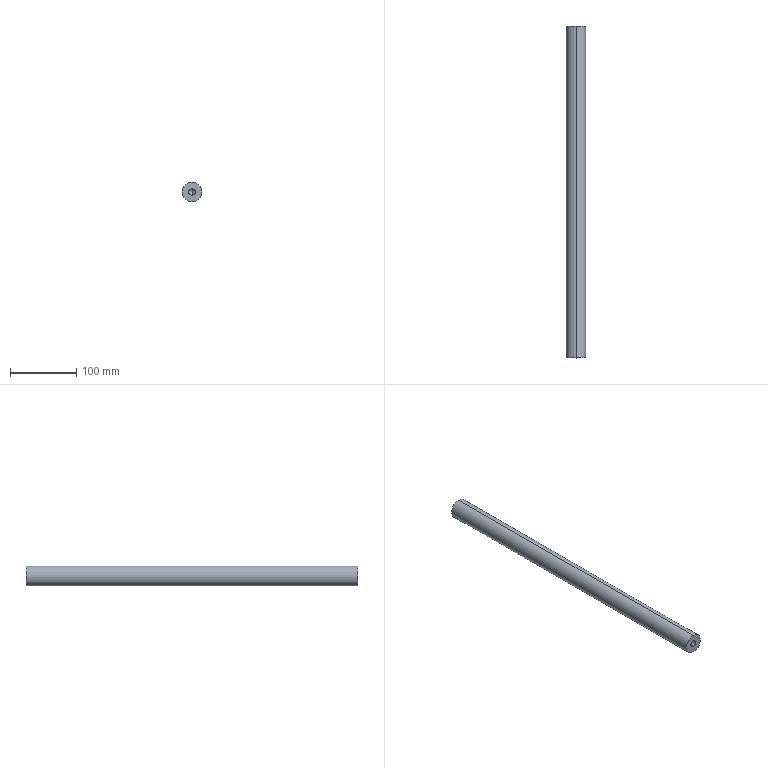Component | SolidWorks | -TopPlateSupport-1 | 1 solid | 12 faces | box 30 x 500 x 30 mm | volume 347910 mm3 | cylinder 6 | cone 4 | plane 2 | commonest cylinder face diameters 10.2 x4 30 x2
build123d program:
from build123d import *

# Parameters (mm, degrees)
SKETCH1_R           = 15
BOSS_EXTRUDE1_DEPTH = 250


with BuildPart() as part:
    # Sketch1 → Boss-Extrude1 (new, symmetric)
    with BuildSketch(Plane(origin=(0, 0, 0), x_dir=(1, 0, 0), z_dir=(0, 1, 0))):
        with Locations(Location((0, 0, 0), (0, 0, 270))):
            Circle(SKETCH1_R)
    extrude(amount=BOSS_EXTRUDE1_DEPTH, both=True)

    # Sketch2 → M12 Tapped Hole1 (revolve, cut)
    with BuildSketch(Plane(origin=(0, 250, 0), x_dir=(0, 0, 1), z_dir=(1, 0, 0))):
        Polygon((0, 0), (0, 35.814), (5.1, 32.75), (5.1, 0), align=None)
    m12_tapped_hole1 = revolve(axis=Axis((0, 256.35, 0), (0, -1, 0)), mode=Mode.SUBTRACT)

    # Mirror1: M12 Tapped Hole1 across plane
    add(m12_tapped_hole1.mirror(Plane.ZX), mode=Mode.SUBTRACT)


solid = part.part

# Placed as in the assembly
solid = solid.moved(Location((130, 1186, -180), (0, 0, 0)))
STEP:
#1=CARTESIAN_POINT('',(5.118,38.14,-6.886));
#2=VERTEX_POINT('',#1);
#3=CARTESIAN_POINT('',(5.118,38.14,-7.287));
#4=VERTEX_POINT('',#3);
#5=CARTESIAN_POINT('',(5.118,38.14,-7.087));
#6=DIRECTION('',(0.,-1.,0.));
#7=DIRECTION('',(0.,0.,-1.));
#8=AXIS2_PLACEMENT_3D('',#5,#6,#7);
#9=CIRCLE('',#8,0.2008);
#10=EDGE_CURVE('',#2,#4,#9,.T.);
#11=ORIENTED_EDGE('',*,*,#10,.F.);
#12=CARTESIAN_POINT('',(5.118,36.85,-6.886));
#13=VERTEX_POINT('',#12);
#14=CARTESIAN_POINT('',(5.118,36.85,-6.886));
#15=DIRECTION('',(0.,-1.,0.));
#16=VECTOR('',#15,39.37);
#17=LINE('',#14,#16);
#18=EDGE_CURVE('',#2,#13,#17,.T.);
#19=ORIENTED_EDGE('',*,*,#18,.T.);
#20=CARTESIAN_POINT('',(5.118,36.85,-7.287));
#21=VERTEX_POINT('',#20);
#22=CARTESIAN_POINT('',(5.118,36.85,-7.087));
#23=DIRECTION('',(0.,-1.,0.));
#24=DIRECTION('',(0.,0.,-1.));
#25=AXIS2_PLACEMENT_3D('',#22,#23,#24);
#26=CIRCLE('',#25,0.2008);
#27=EDGE_CURVE('',#13,#21,#26,.T.);
#28=ORIENTED_EDGE('',*,*,#27,.T.);
#29=CARTESIAN_POINT('',(5.118,36.85,-7.287));
#30=DIRECTION('',(0.,-1.,0.));
#31=VECTOR('',#30,39.37);
#32=LINE('',#29,#31);
#33=EDGE_CURVE('',#4,#21,#32,.T.);
#34=ORIENTED_EDGE('',*,*,#33,.F.);
#35=EDGE_LOOP('',(#11,#19,#28,#34));
#36=FACE_OUTER_BOUND('',#35,.T.);
#37=CARTESIAN_POINT('',(5.118,36.85,-7.087));
#38=DIRECTION('',(0.,-1.,0.));
#39=DIRECTION('',(0.,0.,-1.));
#40=AXIS2_PLACEMENT_3D('',#37,#38,#39);
#41=CYLINDRICAL_SURFACE('',#40,0.2008);
#42=ADVANCED_FACE('',(#36),#41,.F.);
#43=CARTESIAN_POINT('',(5.118,38.26,-7.087));
#44=VERTEX_POINT('',#43);
#45=CARTESIAN_POINT('',(5.118,38.14,-7.287));
#46=DIRECTION('',(0.,-0.515,-0.8572));
#47=VECTOR('',#46,39.37);
#48=LINE('',#45,#47);
#49=EDGE_CURVE('',#44,#4,#48,.T.);
#50=ORIENTED_EDGE('',*,*,#49,.F.);
#51=CARTESIAN_POINT('',(5.118,38.14,-6.886));
#52=DIRECTION('',(0.,-0.515,0.8572));
#53=VECTOR('',#52,39.37);
#54=LINE('',#51,#53);
#55=EDGE_CURVE('',#44,#2,#54,.T.);
#56=ORIENTED_EDGE('',*,*,#55,.T.);
#57=ORIENTED_EDGE('',*,*,#10,.T.);
#58=EDGE_LOOP('',(#50,#56,#57));
#59=FACE_OUTER_BOUND('',#58,.T.);
#60=CARTESIAN_POINT('',(5.118,38.14,-7.087));
#61=DIRECTION('',(0.,-1.,0.));
#62=DIRECTION('',(0.,0.,-1.));
#63=AXIS2_PLACEMENT_3D('',#60,#61,#62);
#64=CONICAL_SURFACE('',#63,0.2008,1.03);
#65=ADVANCED_FACE('',(#59),#64,.F.);
#66=CARTESIAN_POINT('',(5.118,55.246,-7.287));
#67=VERTEX_POINT('',#66);
#68=CARTESIAN_POINT('',(5.118,55.246,-6.886));
#69=VERTEX_POINT('',#68);
#70=CARTESIAN_POINT('',(5.118,55.246,-7.087));
#71=DIRECTION('',(0.,1.,0.));
#72=DIRECTION('',(0.,0.,1.));
#73=AXIS2_PLACEMENT_3D('',#70,#71,#72);
#74=CIRCLE('',#73,0.2008);
#75=EDGE_CURVE('',#67,#69,#74,.T.);
#76=ORIENTED_EDGE('',*,*,#75,.F.);
#77=CARTESIAN_POINT('',(5.118,56.535,-7.287));
#78=VERTEX_POINT('',#77);
#79=CARTESIAN_POINT('',(5.118,56.535,-7.287));
#80=DIRECTION('',(0.,1.,0.));
#81=VECTOR('',#80,39.37);
#82=LINE('',#79,#81);
#83=EDGE_CURVE('',#67,#78,#82,.T.);
#84=ORIENTED_EDGE('',*,*,#83,.T.);
#85=CARTESIAN_POINT('',(5.118,56.535,-6.886));
#86=VERTEX_POINT('',#85);
#87=CARTESIAN_POINT('',(5.118,56.535,-7.087));
#88=DIRECTION('',(0.,1.,0.));
#89=DIRECTION('',(0.,0.,1.));
#90=AXIS2_PLACEMENT_3D('',#87,#88,#89);
#91=CIRCLE('',#90,0.2008);
#92=EDGE_CURVE('',#78,#86,#91,.T.);
#93=ORIENTED_EDGE('',*,*,#92,.T.);
#94=CARTESIAN_POINT('',(5.118,56.535,-6.886));
#95=DIRECTION('',(0.,1.,0.));
#96=VECTOR('',#95,39.37);
#97=LINE('',#94,#96);
#98=EDGE_CURVE('',#69,#86,#97,.T.);
#99=ORIENTED_EDGE('',*,*,#98,.F.);
#100=EDGE_LOOP('',(#76,#84,#93,#99));
#101=FACE_OUTER_BOUND('',#100,.T.);
#102=CARTESIAN_POINT('',(5.118,56.535,-7.087));
#103=DIRECTION('',(0.,1.,0.));
#104=DIRECTION('',(0.,0.,1.));
#105=AXIS2_PLACEMENT_3D('',#102,#103,#104);
#106=CYLINDRICAL_SURFACE('',#105,0.2008);
#107=ADVANCED_FACE('',(#101),#106,.F.);
#108=CARTESIAN_POINT('',(5.118,55.125,-7.087));
#109=VERTEX_POINT('',#108);
#110=CARTESIAN_POINT('',(5.118,55.246,-6.886));
#111=DIRECTION('',(0.,0.515,0.8572));
#112=VECTOR('',#111,39.37);
#113=LINE('',#110,#112);
#114=EDGE_CURVE('',#109,#69,#113,.T.);
#115=ORIENTED_EDGE('',*,*,#114,.F.);
#116=CARTESIAN_POINT('',(5.118,55.246,-7.287));
#117=DIRECTION('',(0.,0.515,-0.8572));
#118=VECTOR('',#117,39.37);
#119=LINE('',#116,#118);
#120=EDGE_CURVE('',#109,#67,#119,.T.);
#121=ORIENTED_EDGE('',*,*,#120,.T.);
#122=ORIENTED_EDGE('',*,*,#75,.T.);
#123=EDGE_LOOP('',(#115,#121,#122));
#124=FACE_OUTER_BOUND('',#123,.T.);
#125=CARTESIAN_POINT('',(5.118,55.246,-7.087));
#126=DIRECTION('',(0.,1.,0.));
#127=DIRECTION('',(0.,0.,1.));
#128=AXIS2_PLACEMENT_3D('',#125,#126,#127);
#129=CONICAL_SURFACE('',#128,0.2008,1.03);
#130=ADVANCED_FACE('',(#124),#129,.F.);
#131=CARTESIAN_POINT('',(5.118,56.535,-6.496));
#132=VERTEX_POINT('',#131);
#133=CARTESIAN_POINT('',(5.118,56.535,-7.677));
#134=VERTEX_POINT('',#133);
#135=CARTESIAN_POINT('',(5.118,56.535,-7.087));
#136=DIRECTION('',(0.,1.,0.));
#137=DIRECTION('',(0.,0.,1.));
#138=AXIS2_PLACEMENT_3D('',#135,#136,#137);
#139=CIRCLE('',#138,0.5906);
#140=EDGE_CURVE('',#132,#134,#139,.T.);
#141=ORIENTED_EDGE('',*,*,#140,.F.);
#142=CARTESIAN_POINT('',(5.118,36.85,-6.496));
#143=VERTEX_POINT('',#142);
#144=CARTESIAN_POINT('',(5.118,56.535,-6.496));
#145=DIRECTION('',(0.,-1.,0.));
#146=VECTOR('',#145,39.37);
#147=LINE('',#144,#146);
#148=EDGE_CURVE('',#132,#143,#147,.T.);
#149=ORIENTED_EDGE('',*,*,#148,.T.);
#150=CARTESIAN_POINT('',(5.118,36.85,-7.677));
#151=VERTEX_POINT('',#150);
#152=CARTESIAN_POINT('',(5.118,36.85,-7.087));
#153=DIRECTION('',(0.,1.,0.));
#154=DIRECTION('',(0.,0.,1.));
#155=AXIS2_PLACEMENT_3D('',#152,#153,#154);
#156=CIRCLE('',#155,0.5906);
#157=EDGE_CURVE('',#143,#151,#156,.T.);
#158=ORIENTED_EDGE('',*,*,#157,.T.);
#159=CARTESIAN_POINT('',(5.118,56.535,-7.677));
#160=DIRECTION('',(0.,-1.,0.));
#161=VECTOR('',#160,39.37);
#162=LINE('',#159,#161);
#163=EDGE_CURVE('',#134,#151,#162,.T.);
#164=ORIENTED_EDGE('',*,*,#163,.F.);
#165=EDGE_LOOP('',(#141,#149,#158,#164));
#166=FACE_OUTER_BOUND('',#165,.T.);
#167=CARTESIAN_POINT('',(5.118,56.535,-7.087));
#168=DIRECTION('',(0.,-1.,0.));
#169=DIRECTION('',(0.,0.,-1.));
#170=AXIS2_PLACEMENT_3D('',#167,#168,#169);
#171=CYLINDRICAL_SURFACE('',#170,0.5906);
#172=ADVANCED_FACE('',(#166),#171,.T.);
#173=ORIENTED_EDGE('',*,*,#148,.F.);
#174=CARTESIAN_POINT('',(5.118,56.535,-7.087));
#175=DIRECTION('',(0.,1.,0.));
#176=DIRECTION('',(0.,0.,1.));
#177=AXIS2_PLACEMENT_3D('',#174,#175,#176);
#178=CIRCLE('',#177,0.5906);
#179=EDGE_CURVE('',#134,#132,#178,.T.);
#180=ORIENTED_EDGE('',*,*,#179,.F.);
#181=ORIENTED_EDGE('',*,*,#163,.T.);
#182=CARTESIAN_POINT('',(5.118,36.85,-7.087));
#183=DIRECTION('',(0.,1.,0.));
#184=DIRECTION('',(0.,0.,1.));
#185=AXIS2_PLACEMENT_3D('',#182,#183,#184);
#186=CIRCLE('',#185,0.5906);
#187=EDGE_CURVE('',#151,#143,#186,.T.);
#188=ORIENTED_EDGE('',*,*,#187,.T.);
#189=EDGE_LOOP('',(#173,#180,#181,#188));
#190=FACE_OUTER_BOUND('',#189,.T.);
#191=CARTESIAN_POINT('',(5.118,56.535,-7.087));
#192=DIRECTION('',(0.,-1.,0.));
#193=DIRECTION('',(0.,0.,-1.));
#194=AXIS2_PLACEMENT_3D('',#191,#192,#193);
#195=CYLINDRICAL_SURFACE('',#194,0.5906);
#196=ADVANCED_FACE('',(#190),#195,.T.);
#197=CARTESIAN_POINT('',(5.118,56.535,-7.087));
#198=DIRECTION('',(0.,1.,0.));
#199=DIRECTION('',(0.,0.,1.));
#200=AXIS2_PLACEMENT_3D('',#197,#198,#199);
#201=CIRCLE('',#200,0.2008);
#202=EDGE_CURVE('',#86,#78,#201,.T.);
#203=ORIENTED_EDGE('',*,*,#202,.F.);
#204=ORIENTED_EDGE('',*,*,#92,.F.);
#205=EDGE_LOOP('',(#203,#204));
#206=FACE_BOUND('',#205,.T.);
#207=ORIENTED_EDGE('',*,*,#179,.T.);
#208=ORIENTED_EDGE('',*,*,#140,.T.);
#209=EDGE_LOOP('',(#207,#208));
#210=FACE_OUTER_BOUND('',#209,.T.);
#211=CARTESIAN_POINT('',(5.118,56.535,-7.087));
#212=DIRECTION('',(0.,1.,0.));
#213=DIRECTION('',(0.,0.,1.));
#214=AXIS2_PLACEMENT_3D('',#211,#212,#213);
#215=PLANE('',#214);
#216=ADVANCED_FACE('',(#206,#210),#215,.T.);
#217=CARTESIAN_POINT('',(5.118,36.85,-7.087));
#218=DIRECTION('',(0.,-1.,0.));
#219=DIRECTION('',(0.,0.,-1.));
#220=AXIS2_PLACEMENT_3D('',#217,#218,#219);
#221=CIRCLE('',#220,0.2008);
#222=EDGE_CURVE('',#21,#13,#221,.T.);
#223=ORIENTED_EDGE('',*,*,#222,.F.);
#224=ORIENTED_EDGE('',*,*,#27,.F.);
#225=EDGE_LOOP('',(#223,#224));
#226=FACE_BOUND('',#225,.T.);
#227=ORIENTED_EDGE('',*,*,#187,.F.);
#228=ORIENTED_EDGE('',*,*,#157,.F.);
#229=EDGE_LOOP('',(#227,#228));
#230=FACE_OUTER_BOUND('',#229,.T.);
#231=CARTESIAN_POINT('',(5.118,36.85,-7.087));
#232=DIRECTION('',(0.,1.,0.));
#233=DIRECTION('',(0.,0.,1.));
#234=AXIS2_PLACEMENT_3D('',#231,#232,#233);
#235=PLANE('',#234);
#236=ADVANCED_FACE('',(#226,#230),#235,.F.);
#237=ORIENTED_EDGE('',*,*,#120,.F.);
#238=ORIENTED_EDGE('',*,*,#114,.T.);
#239=CARTESIAN_POINT('',(5.118,55.246,-7.087));
#240=DIRECTION('',(0.,1.,0.));
#241=DIRECTION('',(0.,0.,1.));
#242=AXIS2_PLACEMENT_3D('',#239,#240,#241);
#243=CIRCLE('',#242,0.2008);
#244=EDGE_CURVE('',#69,#67,#243,.T.);
#245=ORIENTED_EDGE('',*,*,#244,.T.);
#246=EDGE_LOOP('',(#237,#238,#245));
#247=FACE_OUTER_BOUND('',#246,.T.);
#248=CARTESIAN_POINT('',(5.118,55.246,-7.087));
#249=DIRECTION('',(0.,1.,0.));
#250=DIRECTION('',(0.,0.,1.));
#251=AXIS2_PLACEMENT_3D('',#248,#249,#250);
#252=CONICAL_SURFACE('',#251,0.2008,1.03);
#253=ADVANCED_FACE('',(#247),#252,.F.);
#254=ORIENTED_EDGE('',*,*,#83,.F.);
#255=ORIENTED_EDGE('',*,*,#244,.F.);
#256=ORIENTED_EDGE('',*,*,#98,.T.);
#257=ORIENTED_EDGE('',*,*,#202,.T.);
#258=EDGE_LOOP('',(#254,#255,#256,#257));
#259=FACE_OUTER_BOUND('',#258,.T.);
#260=CARTESIAN_POINT('',(5.118,56.535,-7.087));
#261=DIRECTION('',(0.,1.,0.));
#262=DIRECTION('',(0.,0.,1.));
#263=AXIS2_PLACEMENT_3D('',#260,#261,#262);
#264=CYLINDRICAL_SURFACE('',#263,0.2008);
#265=ADVANCED_FACE('',(#259),#264,.F.);
#266=ORIENTED_EDGE('',*,*,#55,.F.);
#267=ORIENTED_EDGE('',*,*,#49,.T.);
#268=CARTESIAN_POINT('',(5.118,38.14,-7.087));
#269=DIRECTION('',(0.,-1.,0.));
#270=DIRECTION('',(0.,0.,-1.));
#271=AXIS2_PLACEMENT_3D('',#268,#269,#270);
#272=CIRCLE('',#271,0.2008);
#273=EDGE_CURVE('',#4,#2,#272,.T.);
#274=ORIENTED_EDGE('',*,*,#273,.T.);
#275=EDGE_LOOP('',(#266,#267,#274));
#276=FACE_OUTER_BOUND('',#275,.T.);
#277=CARTESIAN_POINT('',(5.118,38.14,-7.087));
#278=DIRECTION('',(0.,-1.,0.));
#279=DIRECTION('',(0.,0.,-1.));
#280=AXIS2_PLACEMENT_3D('',#277,#278,#279);
#281=CONICAL_SURFACE('',#280,0.2008,1.03);
#282=ADVANCED_FACE('',(#276),#281,.F.);
#283=ORIENTED_EDGE('',*,*,#18,.F.);
#284=ORIENTED_EDGE('',*,*,#273,.F.);
#285=ORIENTED_EDGE('',*,*,#33,.T.);
#286=ORIENTED_EDGE('',*,*,#222,.T.);
#287=EDGE_LOOP('',(#283,#284,#285,#286));
#288=FACE_OUTER_BOUND('',#287,.T.);
#289=CARTESIAN_POINT('',(5.118,36.85,-7.087));
#290=DIRECTION('',(0.,-1.,0.));
#291=DIRECTION('',(0.,0.,-1.));
#292=AXIS2_PLACEMENT_3D('',#289,#290,#291);
#293=CYLINDRICAL_SURFACE('',#292,0.2008);
#294=ADVANCED_FACE('',(#288),#293,.F.);
#295=CLOSED_SHELL('',(#42,#65,#107,#130,#172,#196,#216,#236,#253,#265,#282,#294));
#296=MANIFOLD_SOLID_BREP('',#295);
#297=CARTESIAN_POINT('',(0.,0.,0.));
#298=DIRECTION('',(0.,0.,1.));
#299=DIRECTION('',(1.,0.,0.));
#300=AXIS2_PLACEMENT_3D('',#297,#298,#299);
#301=(LENGTH_UNIT()NAMED_UNIT(*)SI_UNIT($,.METRE.));
#302=LENGTH_MEASURE_WITH_UNIT(LENGTH_MEASURE(0.0254),#301);
#303=DIMENSIONAL_EXPONENTS(1.,0.,0.,0.,0.,0.,0.);
#304=(CONVERSION_BASED_UNIT('',#302)LENGTH_UNIT()NAMED_UNIT(#303));
#305=UNCERTAINTY_MEASURE_WITH_UNIT(LENGTH_MEASURE(0.00001),#304,'','');
#306=(NAMED_UNIT(*)PLANE_ANGLE_UNIT()SI_UNIT($,.RADIAN.));
#307=(NAMED_UNIT(*)SI_UNIT($,.STERADIAN.)SOLID_ANGLE_UNIT());
#308=(GEOMETRIC_REPRESENTATION_CONTEXT(3)GLOBAL_UNCERTAINTY_ASSIGNED_CONTEXT((#305))GLOBAL_UNIT_ASSIGNED_CONTEXT((#304,#306,#307))REPRESENTATION_CONTEXT('',''));
#309=ADVANCED_BREP_SHAPE_REPRESENTATION('',(#296,#300),#308);
#310=COLOUR_RGB('',0.7922,0.8196,0.9333);
#311=FILL_AREA_STYLE_COLOUR('',#310);
#312=FILL_AREA_STYLE('',(#311));
#313=SURFACE_STYLE_FILL_AREA(#312);
#314=SURFACE_SIDE_STYLE('',(#313));
#315=SURFACE_STYLE_USAGE(.BOTH.,#314);
#316=PRESENTATION_STYLE_ASSIGNMENT((#315));
#317=STYLED_ITEM('',(#316),#296);
#318=(LENGTH_UNIT()NAMED_UNIT(*)SI_UNIT($,.METRE.));
#319=LENGTH_MEASURE_WITH_UNIT(LENGTH_MEASURE(0.0254),#318);
#320=DIMENSIONAL_EXPONENTS(1.,0.,0.,0.,0.,0.,0.);
#321=(CONVERSION_BASED_UNIT('',#319)LENGTH_UNIT()NAMED_UNIT(#320));
#322=UNCERTAINTY_MEASURE_WITH_UNIT(LENGTH_MEASURE(0.00001),#321,'','');
#323=(NAMED_UNIT(*)PLANE_ANGLE_UNIT()SI_UNIT($,.RADIAN.));
#324=(NAMED_UNIT(*)SI_UNIT($,.STERADIAN.)SOLID_ANGLE_UNIT());
#325=(GEOMETRIC_REPRESENTATION_CONTEXT(3)GLOBAL_UNCERTAINTY_ASSIGNED_CONTEXT((#322))GLOBAL_UNIT_ASSIGNED_CONTEXT((#321,#323,#324))REPRESENTATION_CONTEXT('',''));
#326=MECHANICAL_DESIGN_GEOMETRIC_PRESENTATION_REPRESENTATION('',(#317),#325);
#327=PRESENTATION_LAYER_ASSIGNMENT('','',(#317));